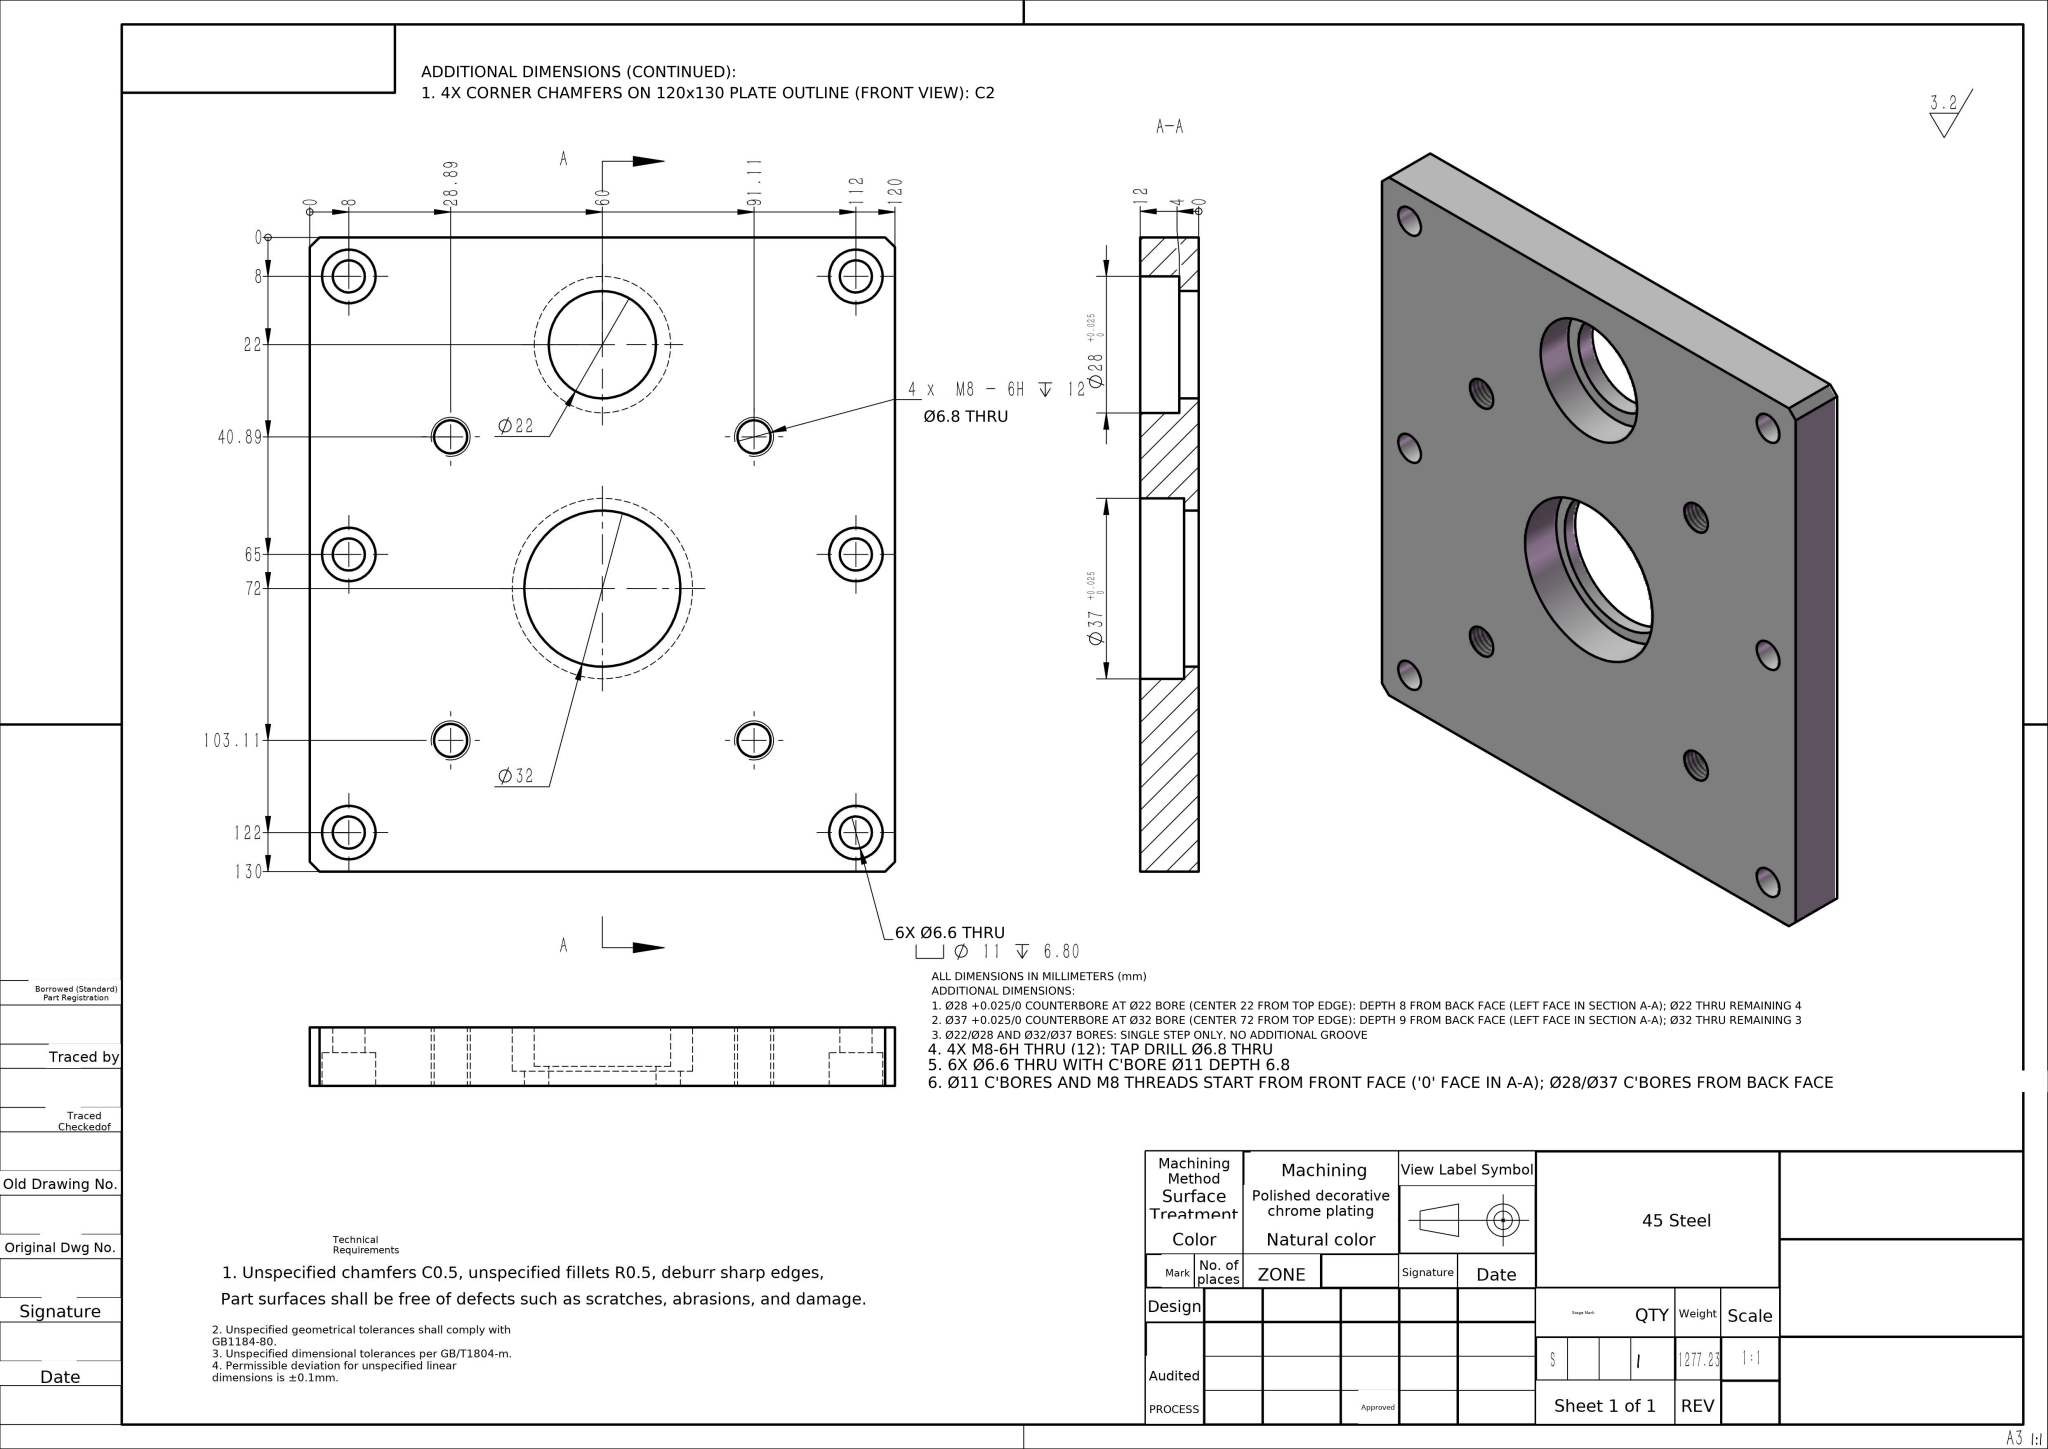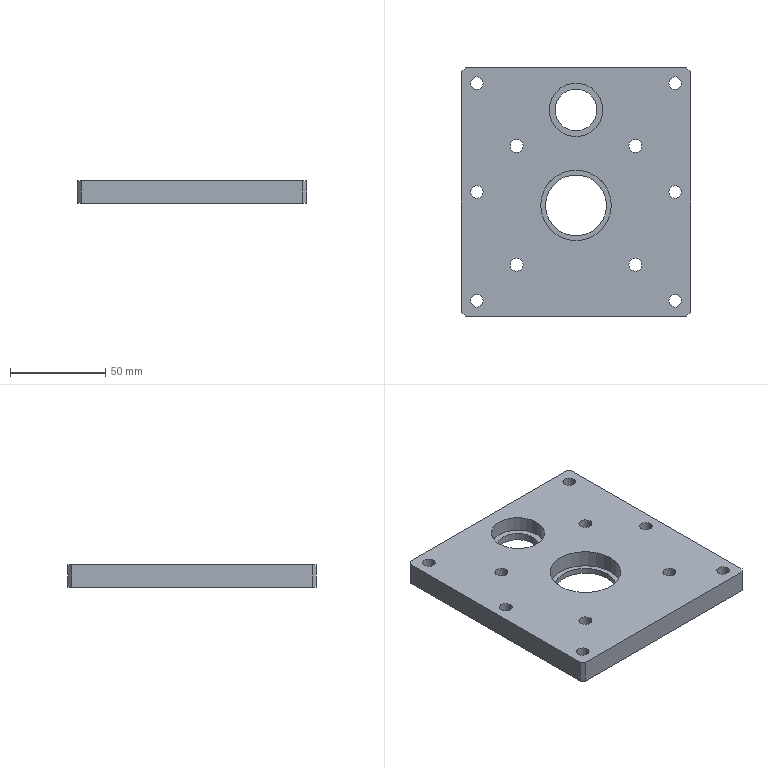Part | NX | mm | 1 solid | 58 faces | box 120 x 130 x 12 mm | volume 161880 mm3 | cylinder 40 | plane 18 | commonest cylinder face diameters 11 x12 6.6 x12 6.8 x8 28 x2 37 x2 32 x2 22 x2